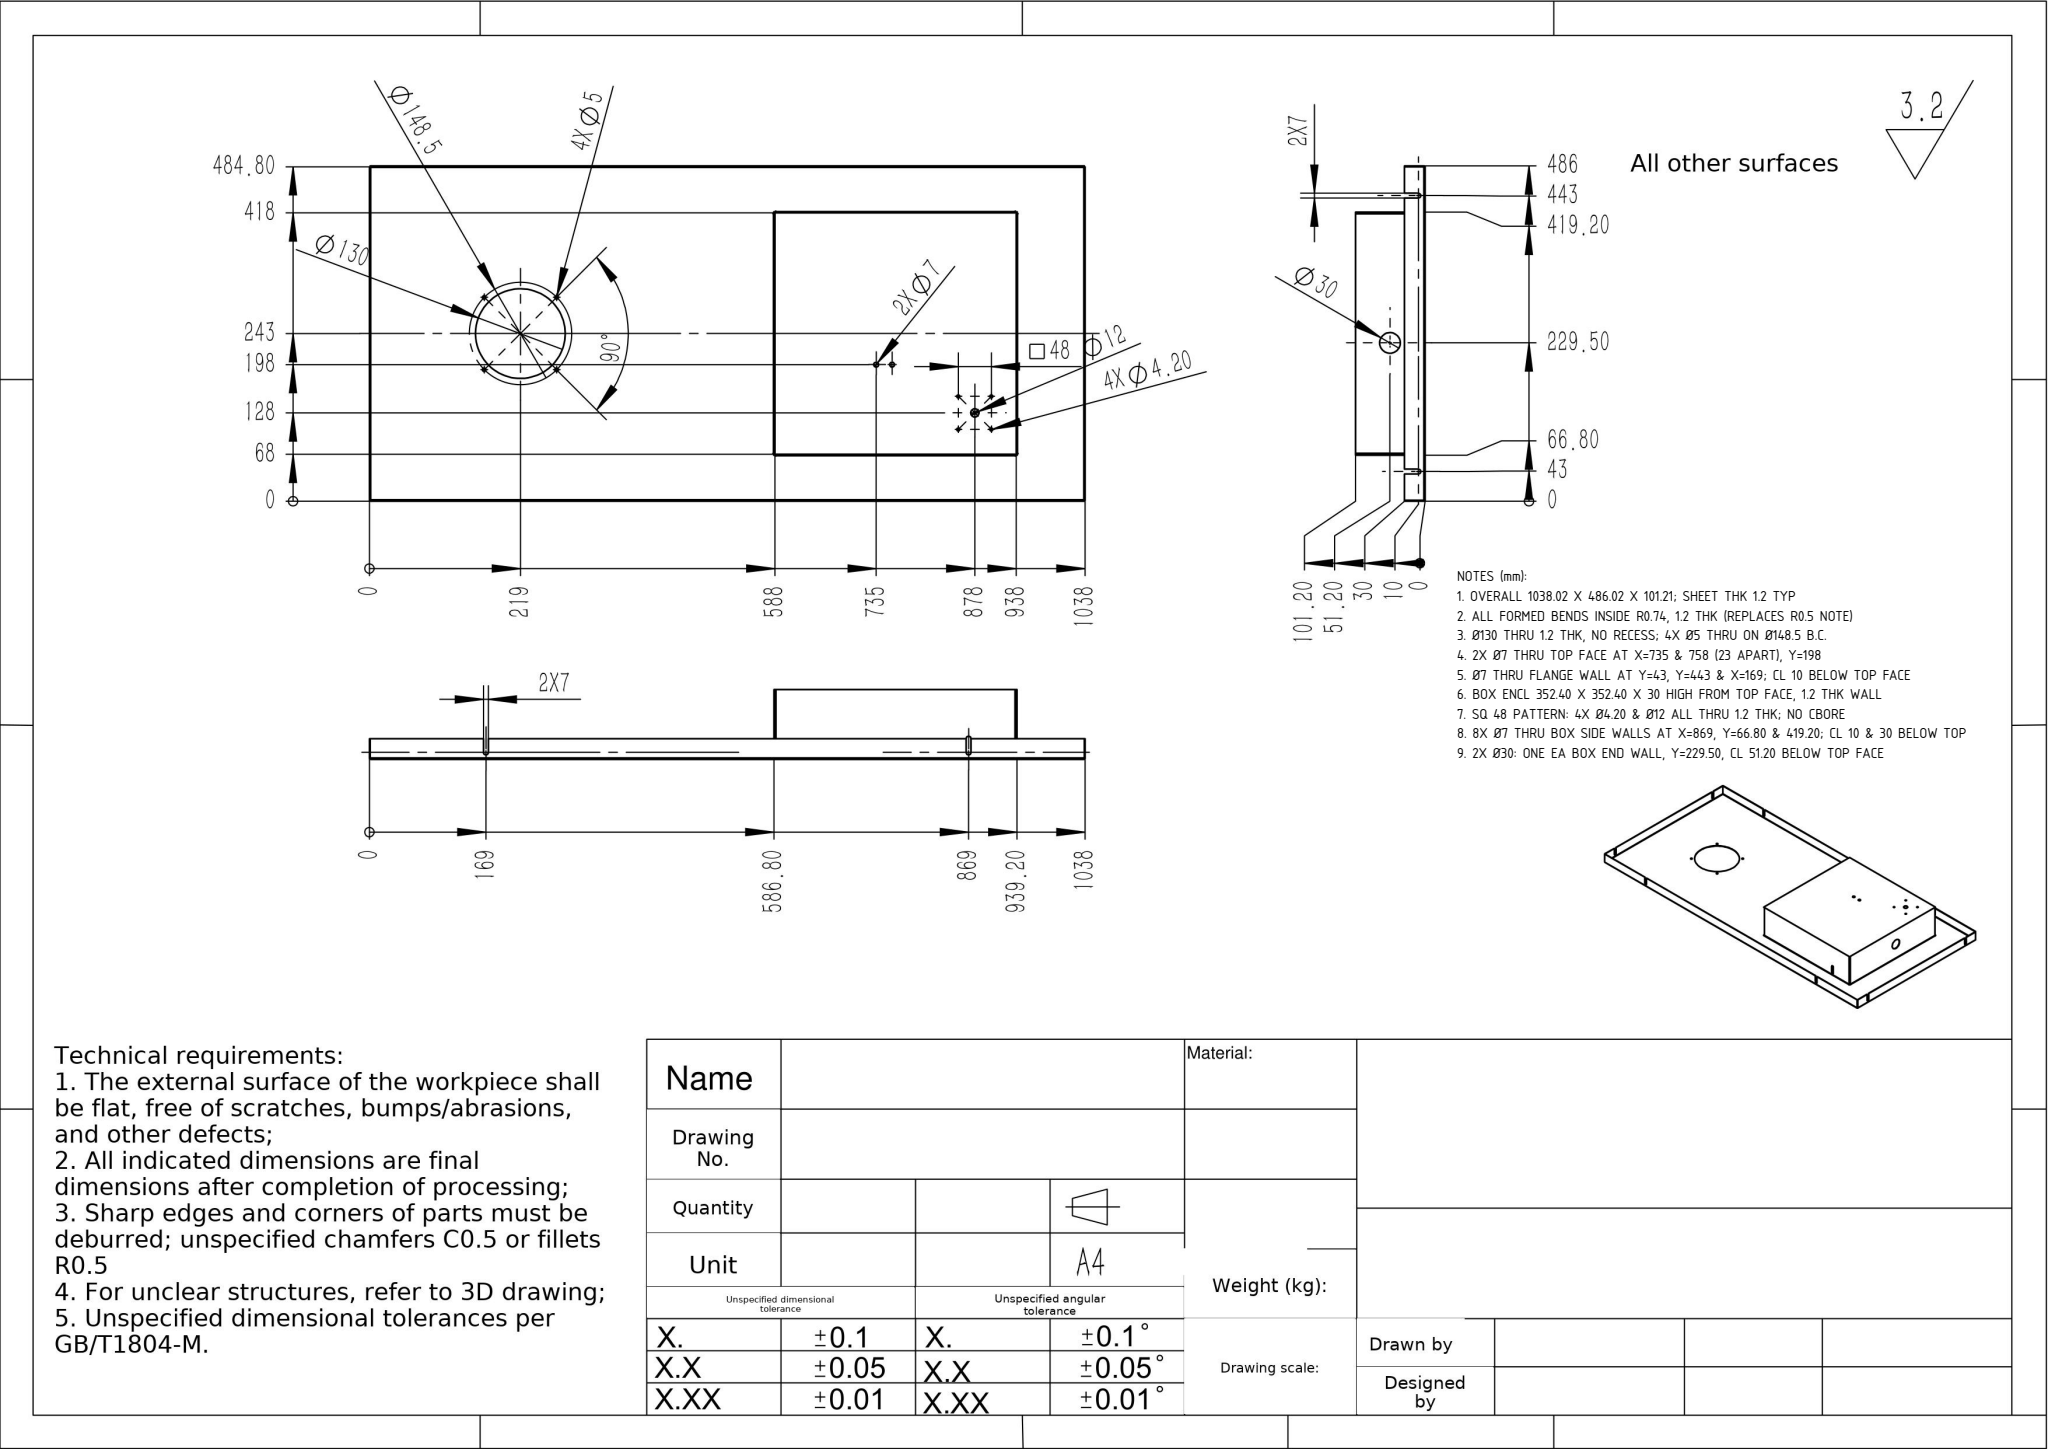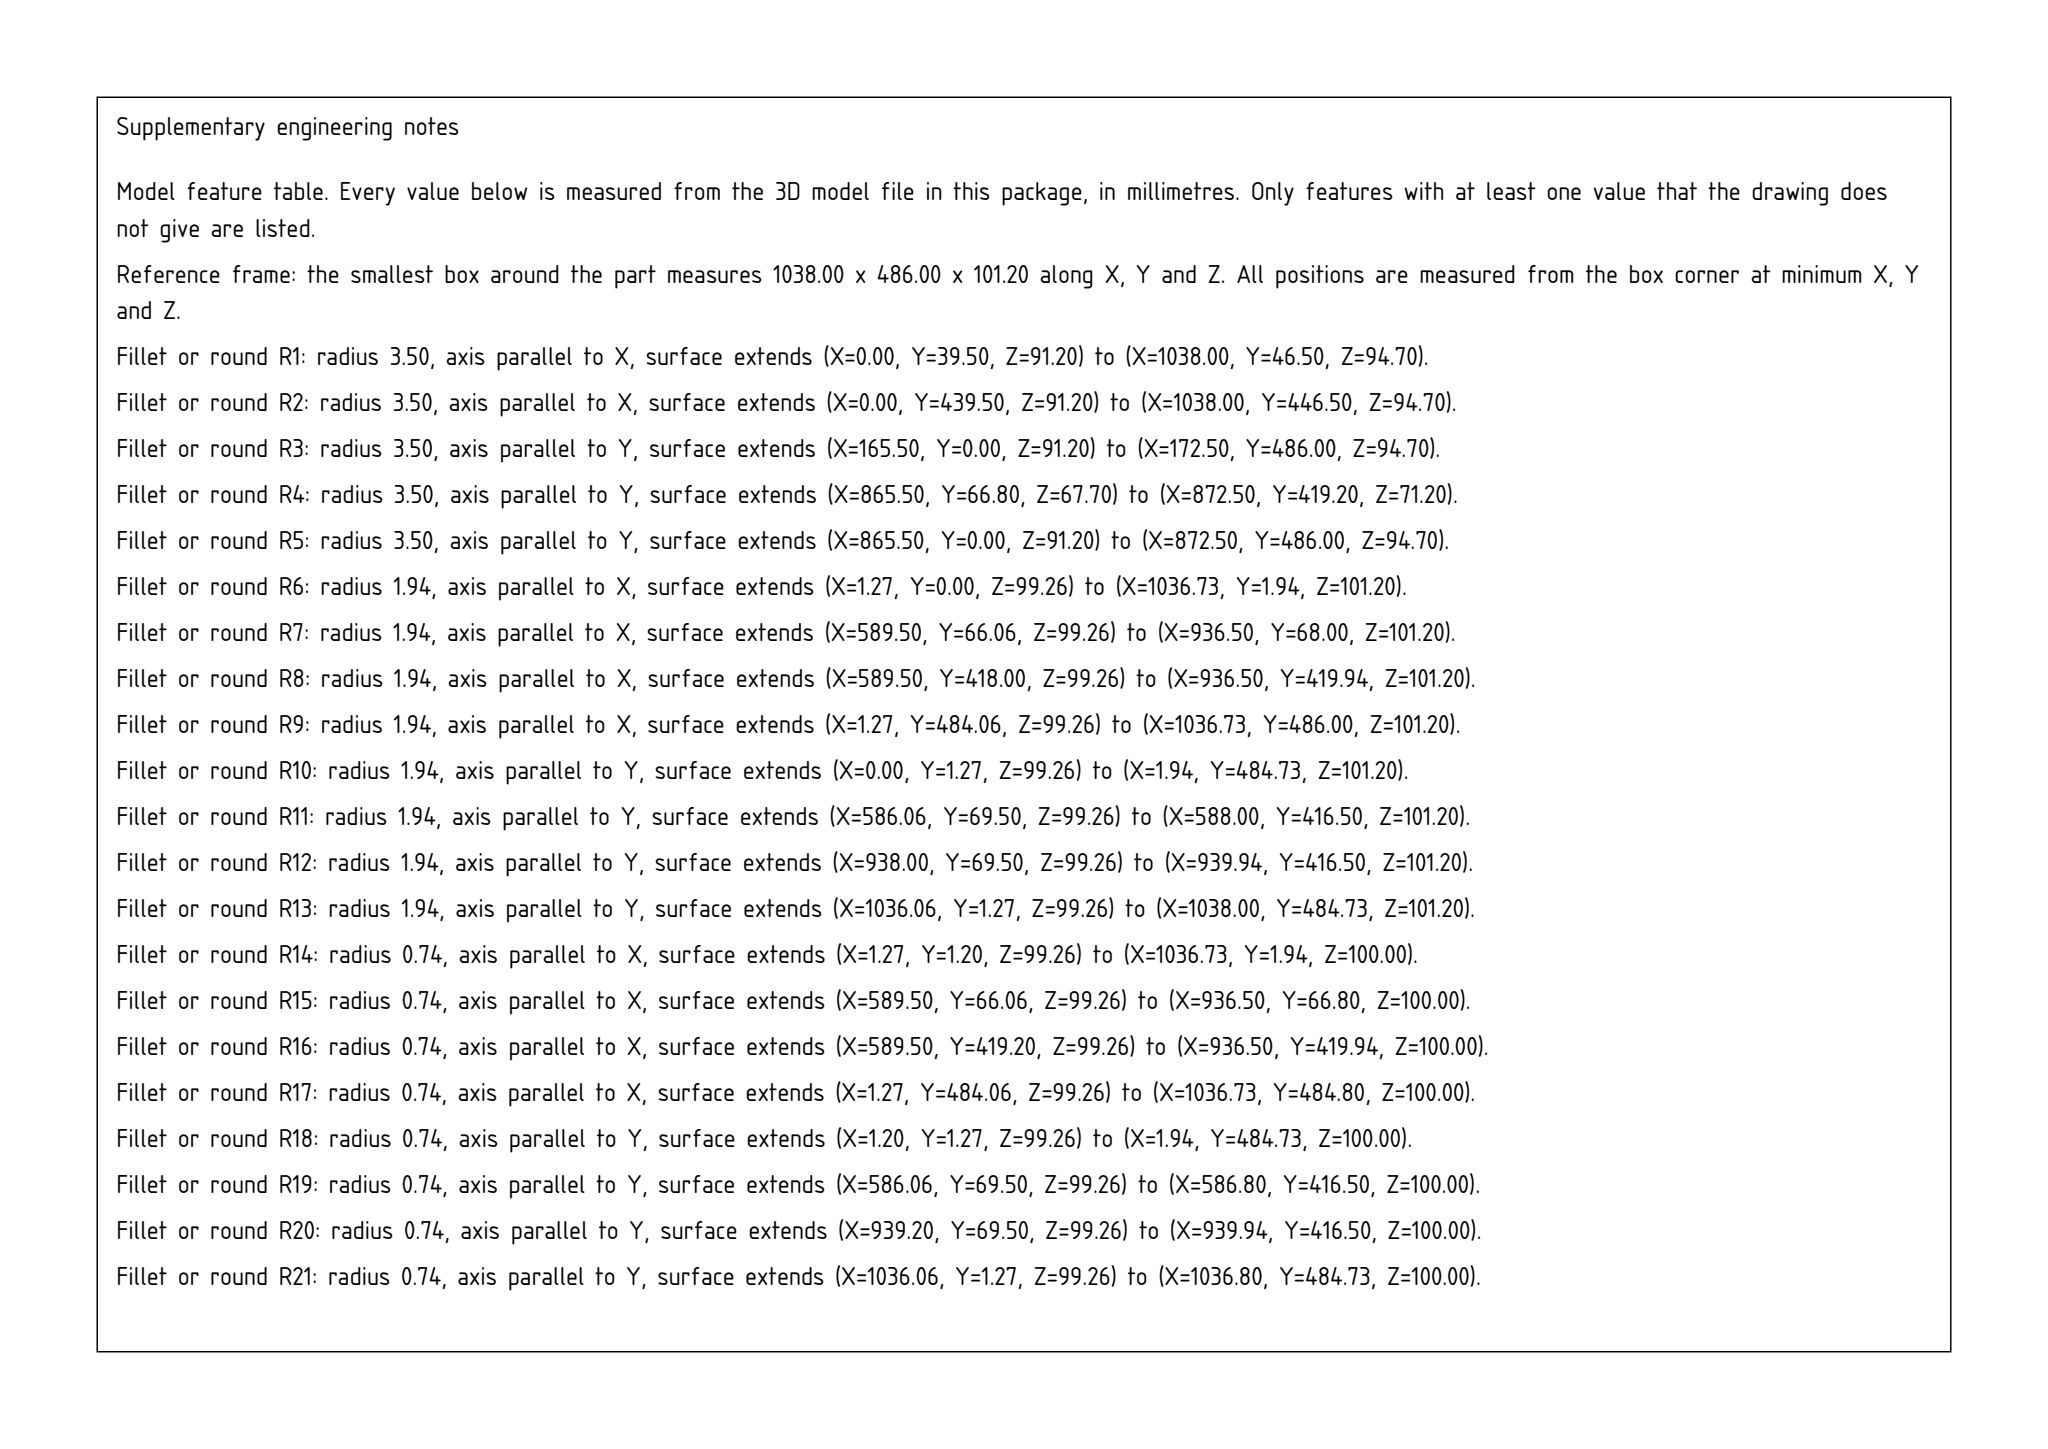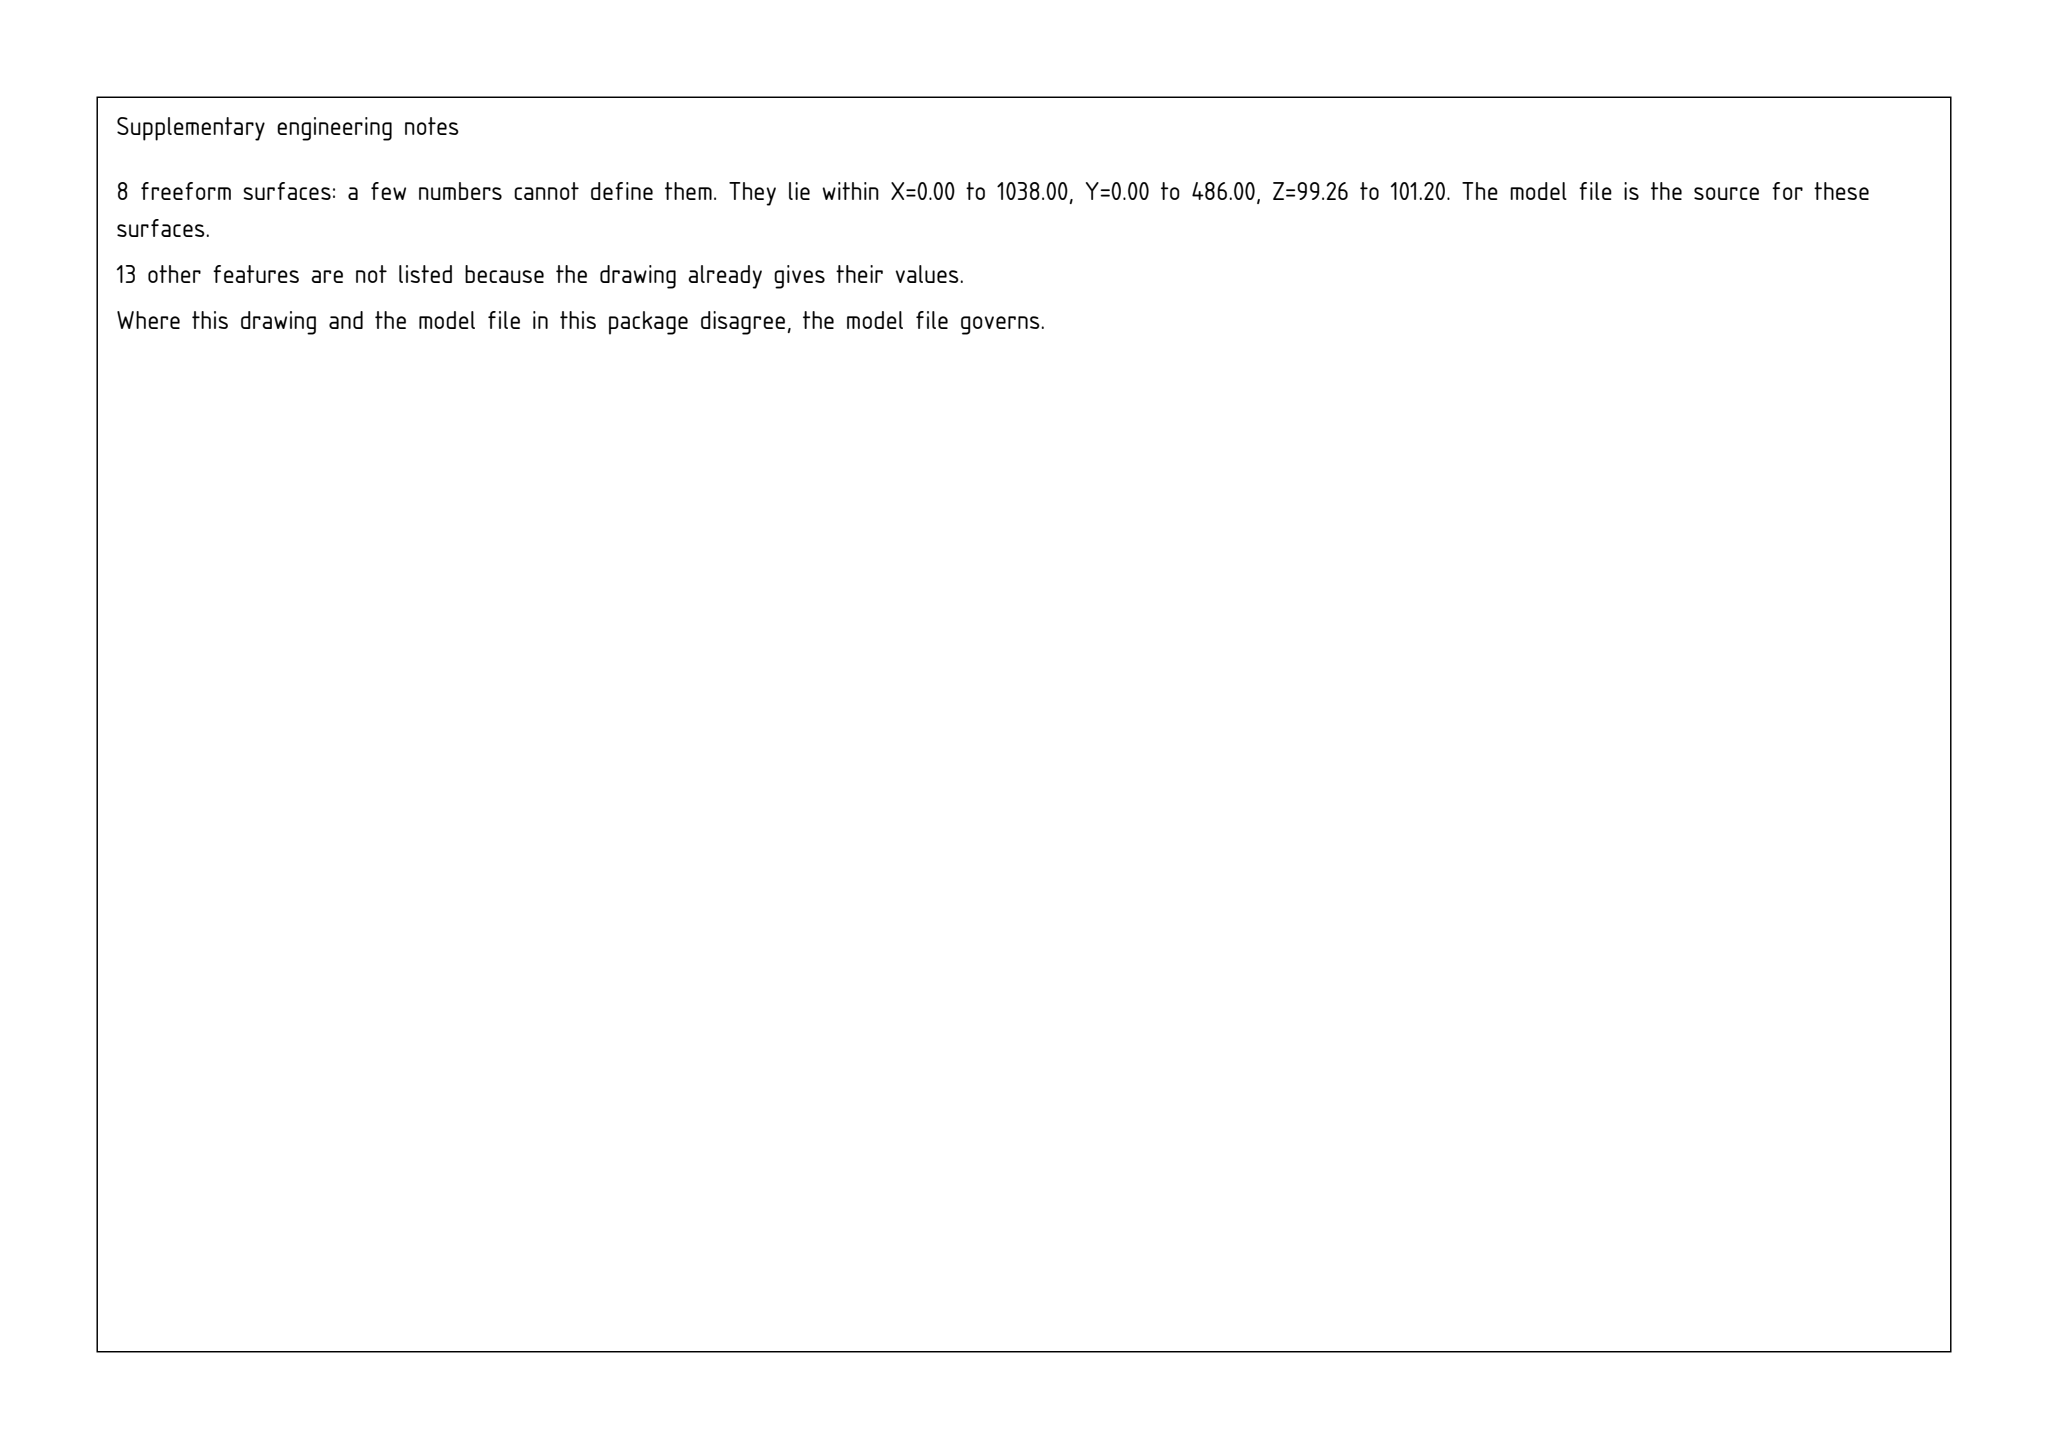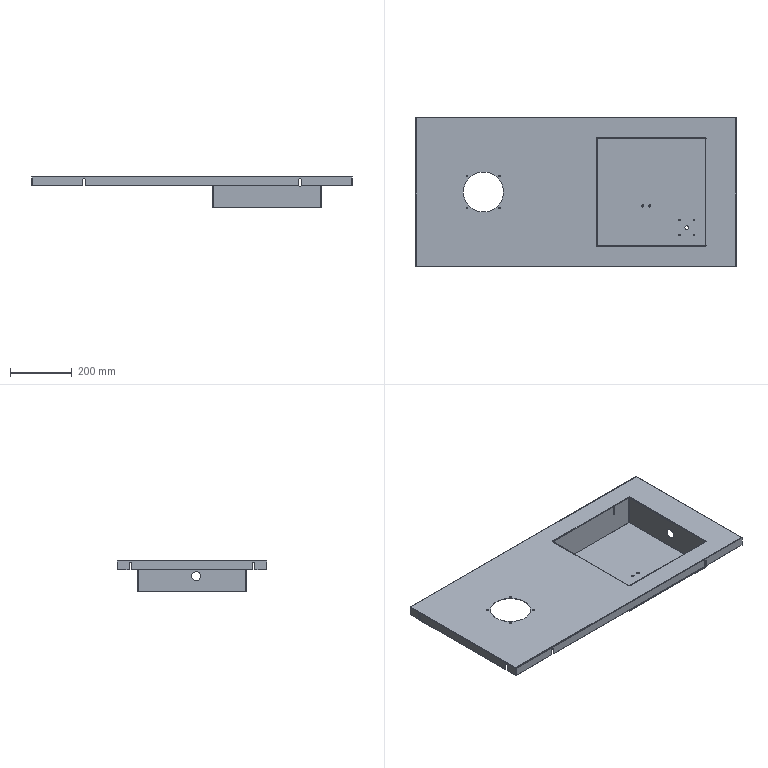Part | SolidWorks | mm | 1 solid | 174 faces | box 1038 x 486 x 101.2 mm | volume 853866 mm3 | plane 108 | cylinder 58 | spline 8 | commonest cylinder face diameters 7 x18 4.2 x8 5 x8 3.873 x8 1.473 x8 30 x4 12 x2 130 x2
Drawing notes:
OVERALL 1038.02 X 486.02 X 101.21; SHEET THK 1.2 TYP | from the solid: bbox_xyz 1038.024/486.024/101.212; faces z=100.0 & 101.2 give 1.2 thk
ALL FORMED BENDS INSIDE R0.74, 1.2 THK (REPLACES R0.5 NOTE) | from the solid: Bend cyls dia 1.473 (R0.7365) inner / 3.873 outer, axes z=99.26 on all perimeter and box edges
Ø130 THRU 1.2 THK, NO RECESS; 4X Ø5 THRU ON Ø148.5 B.C. | from the solid: Cyl dia 130 axis z at (219.01,243.01) L=1.2; 4X dia 5 at (166.51/271.51,190.51/295.51) L=1.2, diag 105√2=148.49
2X Ø7 THRU TOP FACE AT X=735 & 758 (23 APART), Y=198 | from the solid: cyls dia 7.0 axis z at [735.01,198.01] and [758.01,198.01], L=1.2
Ø7 THRU FLANGE WALL AT Y=43, Y=443 & X=169; CL 10 BELOW TOP FACE | from the solid: Cyls dia 7 axis x at y=43.01 & 443.01, axis y at x=169.01, all z=91.2, L=1.2; top face z=101.2
BOX ENCL 352.40 X 352.40 X 30 HIGH FROM TOP FACE, 1.2 THK WALL | from the solid: Outer planes x=586.81/939.21, y=66.81/419.21; inner 588.01/938.01, 68.01/418.01; floor z=71.2 vs top z=101.2
SQ 48 PATTERN: 4X Ø4.20 & Ø12 ALL THRU 1.2 THK; NO CBORE | from the solid: Dia 4.20 at (854.01/902.01,104.01/152.01) and dia 12 at (878.01,128.01), axis z, L=1.2; 48 spacing
8X Ø7 THRU BOX SIDE WALLS AT X=869, Y=66.80 & 419.20; CL 10 & 30 BELOW TOP | from the solid: Dia 7 y-axis at x=869.01: 4 at z=91.2 + 4 at z=71.2; walls y=66.81/68.01 and 418.01/419.21; 101.2-91.2=10, 101.2-71.2=30
2X Ø30: ONE EA BOX END WALL, Y=229.50, CL 51.20 BELOW TOP FACE | from the solid: Dia 30 x-axis cyls, y=229.51, z=50.0, count 4 (2 wall layers ea end); end walls x=586.81/588.01 and 938.01/939.21